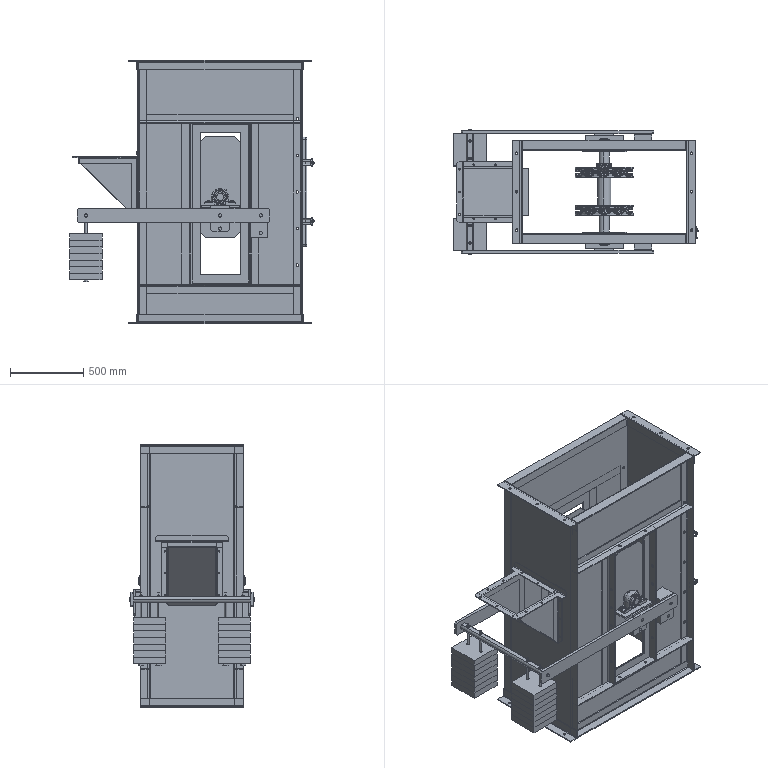Assembly | SolidWorks | mm | 60 component files | 82 solids | 3008 faces | box 1670 x 856 x 1800 mm | volume 98350600 mm3 | plane 1018 | cylinder 784 | cone 482 | sphere 288 | torus 282 | spline 154 | commonest cylinder face diameters 18 x195 20 x67 12 x62 367 x52 9 x40 10 x34 22 x32 60 x24
Bill of materials:
AccessDoor | 1 |  | Thin rectangular panel with rounded corners and edges, with two eyelet tabs sticking out from one long edge and two small hooked/slotted tabs on the face near the opposite edge.
ConnectingRod | 2 |  | Long, flat rectangular bar with chamfered corners and three small through holes along its centerline, spaced unevenly.
Counterweight | 14 |  | Square, fairly thick plate or block with two round through holes on one centerline.
FixedFrame | 1 |  | Long shaft with two parallel flats along its main body, smaller round journals at both ends, and four radial holes through the flat face.
GB_T62.1-2004WingNutRoundWingM12_1.75 | 2 |  | Bent bracket or lug with a central cylindrical boss with a through bore, and two angled arms that end in rounded eyelets with holes.
GuideFrame_2 | 2 |  | Open rectangular frame made of flat-bar members set on edge, with small holes along its sides and ends.
HangerRod | 4 |  | Long, slender cylindrical rod with a thin hexagonal head at one end and a short, smaller-diameter stepped pin at the other end.
hex nuts 1-fine pitch-grades ab gb | 8 |  | Hexagonal nut-shaped block with a central round through bore and chamfered corners on both faces.
Inlet | 1 |  | Sheet-metal chute or hopper: a rectangular flanged inlet frame with bolt holes, a sloped bottom wall, triangular side walls, and flanged side strips with holes.
LinkBolt | 2 |  | Lever-type part: a short cylindrical ring boss with a through bore and a straight cylindrical arm sticking out sideways, ending in a chamfered tip.
LowerCasing | 1 |  | Sheet-metal rectangular box housing with flanged top and bottom openings that have bolt holes, inner reinforcing channels or ribs, a rectangular side window, a rectangular opening in the back panel, and small lugs and a small block attached.
curved single coil spring lock washers gb | 4 |  | Flat split ring with a rectangular cross-section and a single radial gap.
DriveSprocket-Driven2 | 1 |  | Disc-shaped wheel with a groove around the rim, a raised central hub with a keyed bore, and six round lightening holes in a ring around the web; resembles a grooved pulley or sheave.
DriveSprocket-DrivenWithBearingHole2 | 1 |  | Disc-shaped grooved wheel almost identical to the keyed variant, but with a plain round central bore inside a raised hub, and six round holes in the web.
GB_T276-94[DeepGrooveBallBearing61914-2Z]2 | 2 |  | Flat annular part made of an outer ring and an inner ring separated by a narrow gap that holds evenly spaced small elements; resembles a thin-section rolling bearing.
GB_T7810-1995BearingWithVerticalSeatUELP210 | 2 |  | Housing on a pedestal base: a rectangular base with two elongated mounting holes supports a rounded, arch-shaped housing. The housing holds a ring insert with a round bore, and a small nipple-like stub sits on top; resembles a pillow-block bearing unit.
GB_T812-1988[RoundNutM68_2] | 2 |  | Flat thick ring with four rectangular notches evenly spaced around the outer edge and chamfered outer edges; resembles a slotted ring nut or locknut.
GB858-1988[LockWasherForRoundNut68_1.5]-Driven2 | 1 |  | Thin flat washer-like ring with one tab pointing inward from the bore edge and several rectangular tabs pointing outward around the outer edge. Some outer tabs are bent out of plane; resembles a tab lock washer.
GuideFrame | 2 |  | L-shaped (angle) bracket of flat plate: a wide horizontal flange with two round holes, joined at right angles to a narrower leg with two round holes and chamfered free corners.
hexagon head bolts--product grade c gb | 4 |  | Hexagon-head fastener-like part: a hexagonal head with a round bearing face and a plain cylindrical shank with a chamfered end; resembles a hex bolt or screw.
LowerAxis | 1 |  | Stepped cylindrical shaft with a larger central section and several smaller-diameter steps toward each end, plus a possible keyway or flat on one step.
ProtectivePlate | 2 |  | Very thin flat rectangular plate with chamfered corners and one central round hole; resembles a shim or spacer plate.
Mates:
1. coincident | LowerCasing-1 face at (-563, -290, 900) dir (-1, 0, 0) | Inlet-1 face at (-563, -163, -195) dir (1, 0, 0)
2. parallel | LowerCasing-1 face at (-563, -290, 900) dir (0, -1, 0) | Inlet-1 face at (-762, -163, 240) dir (0, -1, 0)
3. parallel | ConnectingRod-1 face at (-977, -398, -110) dir (0, 0, 1) | ConnectingRod-2 face at (-977, 418, -110) dir (0, 0, 1)
4. concentric | ConnectingRod-1 face at (-917, -398, -160) dir (0, -1, 0) r 11 | ConnectingRod-2 face at (-917, 418, -160) dir (0, -1, 0) r 11
5. width | ConnectingRod-1 face at (-319.5, -418, -160) dir (0, -1, 0) | ConnectingRod-2 face at (-319.5, 418, -160) dir (0, 1, 0) | LowerCasing-1 face at (-563, 290, 900) dir (0, 1, 0) | LowerCasing-1 face at (-563, -290, 900) dir (0, -1, 0)
6. distance | ConnectingRod-2 face at (-319.5, 398, -160) dir (0, -1, 0) | ConnectingRod-1 face at (-319.5, -398, -160) dir (0, 1, 0)
7. parallel | LowerCasing-1 face at (-652.095, -290, -630) dir (0, 0, 1) | ConnectingRod-1 face at (-977, -398, -110) dir (0, 0, 1)
8. distance | ConnectingRod-1 sketch segment at (278, -409.25, -160) dir (0, -1, 0) | LowerCasing-1 face at (563, -290, 900) dir (1, 0, 0)
9. distance | ConnectingRod-1 sketch segment at (278, -409.25, -160) dir (0, -1, 0) | LowerCasing-1 face at (563, 353, -900) dir (0, 0, -1)
10. concentric | ConnectingRod-2 face at (-917, 418, -160) dir (0, -1, 0) r 11 | FixedFrame-1 face at (-917, -428, -160) dir (0, 1, 0) r 11
11. coincident | ConnectingRod-1 face at (-319.5, -398, -160) dir (0, 1, 0) | FixedFrame-1 face at (-917, -398, -160) dir (0, -1, 0)
12. parallel | ConnectingRod-2 face at (-977, 418, -110) dir (0, 0, 1) | FixedFrame-1 face at (-947, 428, -140) dir (0, 0, 1)
13. concentric | FixedFrame-1 face at (-917, 348, -796) dir (0, 0, 1) r 9 | HangerRod-1 face at (-917, 348, -115) dir (0, 0, -1) r 8
14. distance | HangerRod-1 face at (-917, 348, -115) dir (0, 0, 1) | FixedFrame-1 face at (-947, 428, -140) dir (0, 0, 1)
15. concentric | FixedFrame-1 face at (-917, 228, -796) dir (0, 0, 1) r 9 | HangerRod-2 face at (-917, 228, -115) dir (0, 0, -1) r 8
16. coincident | HangerRod-1 face at (-917, 348, -115) dir (0, 0, 1) | HangerRod-2 face at (-917, 228, -115) dir (0, 0, 1)
17. concentric | Counterweight-1 face at (-917, 348, -555) dir (0, 0, -1) r 10 | HangerRod-1 face at (-917, 348, -115) dir (0, 0, -1) r 8
18. concentric | Counterweight-1 edge at (-917, 228, -555) dir (0, 0, 1) r 10 | HangerRod-2 face at (-917, 228, -115) dir (0, 0, -1) r 8
19. coincident | Counterweight-1 face at (-917, 288, -600) dir (0, 0, -1) | HangerRod-1 face at (-917, 348, -600) dir (0, 0, 1)
20. concentric | FixedFrame-1 face at (-917, 228, -796) dir (0, 0, 1) r 9 | hex nuts 1-fine pitch-grades ab gb-2 face at (-917, 228, -140) dir (0, 0, 1) r 523.599
21. coincident | FixedFrame-1 face at (-947, 428, -140) dir (0, 0, 1) | hex nuts 1-fine pitch-grades ab gb-2 face at (-930.856, 220, -140) dir (0, 0, -1)
22. concentric | FixedFrame-1 face at (-917, 348, -796) dir (0, 0, 1) r 9 | hex nuts 1-fine pitch-grades ab gb-3 face at (-917, 348, -140) dir (0, 0, 1) r 523.599
23. coincident | FixedFrame-1 face at (-947, 428, -140) dir (0, 0, 1) | hex nuts 1-fine pitch-grades ab gb-3 face at (-930.856, 340, -140) dir (0, 0, -1)
24. coincident | LowerCasing-1 face at (-652.095, -290, -630) dir (0, 0, 1) | GuideFrame_2-1 face at (-200, -353, -630) dir (0, 0, -1)
25. coincident | LowerCasing-1 face at (200, -353, -500000) dir (-1, 0, 0) | GuideFrame_2-1 face at (200, -353, -630) dir (1, 0, 0)
26. coincident | LowerCasing-1 face at (-563, -290, 900) dir (0, -1, 0) | GuideFrame_2-1 face at (0, -290, -80) dir (0, 1, 0)
27. concentric | LowerTensioningDeviceAssembly-1/GuideFrame-2 face at (0, -398, -160) dir (0, 1, 0) r 11 | ConnectingRod-1 face at (0, -398, -160) dir (0, -1, 0) r 11
28. coincident | LowerTensioningDeviceAssembly-1/GuideFrame-2 face at (65, -398, -95) dir (0, -1, 0) | ConnectingRod-1 face at (-319.5, -398, -160) dir (0, 1, 0)
29. perpendicular | LowerTensioningDeviceAssembly-1/GuideFrame-1 face at (-65, 74, -270) dir (-1, 0, 0) | ConnectingRod-2 face at (-977, 418, -110) dir (0, 0, 1)
30. coincident | LowerCasing-1 face at (563, -290, 900) dir (1, 0, 0) | AccessDoor-1 face at (563, -269, -357) dir (-1, 0, 0)
31. parallel | LowerCasing-1 edge at (563, -200, 350) dir (0, 0, -1) | AccessDoor-1 edge at (563, -289, 357) dir (0, 0, -1)
32. width | AccessDoor-1 face at (563, -269, 377) dir (0.1736, 0, 0.9848) | AccessDoor-1 face at (563, -269, -377) dir (0.1736, 0, -0.9848) | LowerCasing-1 face at (553, -200, 350) dir (0, 0, -1) | LowerCasing-1 face at (553, -200, -350) dir (0, 0, 1)
33. width | AccessDoor-1 face at (563, -289, -357) dir (0.1736, -0.9848, 0) | AccessDoor-1 face at (563, 289, -357) dir (0.1736, 0.9848, 0) | LowerCasing-1 face at (553, -200, 350) dir (0, 1, 0) | LowerCasing-1 face at (553, 200, 350) dir (0, -1, 0)
34. concentric | AccessDoor-1 face at (628, -219, 200) dir (0, -1, 0) r 6.5 | LinkBolt-1 face at (628, -243, 200) dir (0, -1, 0) r 6
35. concentric | LowerCasing-1 face at (628, -313, 205) dir (0, 0, -1) r 5 | LinkBolt-1 face at (628, -313, 207) dir (0, 0, -1) r 8
36. concentric | LowerCasing-1 face at (628, -313, -205) dir (0, 0, 1) r 5 | LinkBolt-2 face at (628, -313, -193) dir (0, 0, -1) r 8
37. concentric | AccessDoor-1 face at (628, -219, -200) dir (0, -1, 0) r 6.5 | LinkBolt-2 face at (628, -243, -200) dir (0, -1, 0) r 6
38. concentric | LinkBolt-1 face at (628, -243, 200) dir (0, -1, 0) r 6 | GB_T62.1-2004WingNutRoundWingM12_1.75-1 face at (628, -234, 200) dir (0, -1, 0) r 6
39. coincident | AccessDoor-1 face at (643, -261, 215) dir (0, 1, 0) | GB_T62.1-2004WingNutRoundWingM12_1.75-1 face at (628, -261, 200) dir (0, -1, 0)
40. concentric | LinkBolt-2 face at (628, -243, -200) dir (0, -1, 0) r 6 | GB_T62.1-2004WingNutRoundWingM12_1.75-2 face at (628, -234, -200) dir (0, -1, 0) r 6
41. coincident | AccessDoor-1 face at (643, -261, -215) dir (0, 1, 0) | GB_T62.1-2004WingNutRoundWingM12_1.75-2 face at (628, -261, -200) dir (0, -1, 0)
42. parallel | LowerCasing-1 face at (563, -290, 989.095) dir (1, 0, 0) | GB_T62.1-2004WingNutRoundWingM12_1.75-2 face at (626, -242.5, -220.5) dir (-1, 0, 0)
43. parallel | LowerCasing-1 face at (563, -290, 989.095) dir (1, 0, 0) | GB_T62.1-2004WingNutRoundWingM12_1.75-1 face at (626, -242.5, 179.5) dir (-1, 0, 0)
44. concentric | LowerCasing-1 face at (-300, -263, 900) dir (0, 0, -1) r 9 | assembly face at (-300, -263, 927) dir (0, 0, -1) r 8
45. coincident | LowerCasing-1 face at (652.095, -303, 892) dir (0, 0, -1) | assembly face at (-288.165, -269.833, 892) dir (0, 0, 1)
46. concentric | LowerCasing-1 face at (-598, -263, 900) dir (0, 0, -1) r 9 | assembly face at (-598, -263, 916) dir (0, 0, 1) r 8
47. coincident | LowerCasing-1 face at (-626, 353, 894) dir (0, 0, -1) | assembly face at (-598, -263, 894) dir (0, 0, 1)
48. coincident | LowerCasing-1 face at (652.095, -303, 892) dir (0, 0, -1) | assembly face at (-300, -263, 892) dir (0, 0, 1)
49. coincident | assembly face at (-300, -263, 869) dir (0, 0, -1) | assembly face at (0, -263, 869) dir (0, 0, -1)
50. coincident | assembly face at (0, -263, 869) dir (0, 0, -1) | assembly face at (300, -263, 869) dir (0, 0, -1)
51. concentric | LowerCasing-1 face at (598, -263, 900) dir (0, 0, -1) r 9 | assembly face at (598, -263, 914) dir (0, 0, 1) r 8
52. coincident | assembly face at (300, -263, 869) dir (0, 0, -1) | assembly face at (598, -263, 869) dir (0, 0, -1)
53. concentric | LowerCasing-1 face at (598, 0, 900) dir (0, 0, -1) r 9 | assembly face at (598, 0, 914) dir (0, 0, 1) r 8
54. coincident | assembly face at (598, -263, 869) dir (0, 0, -1) | assembly face at (598, 0, 869) dir (0, 0, -1)
55. concentric | LowerCasing-1 face at (598, 263, 900) dir (0, 0, -1) r 9 | assembly face at (598, 263, 914) dir (0, 0, 1) r 8
56. coincident | assembly face at (598, 263, 869) dir (0, 0, -1) | assembly face at (598, 0, 869) dir (0, 0, -1)
57. concentric | LowerCasing-1 face at (-598, 263, 900) dir (0, 0, -1) r 9 | assembly face at (-598, 263, 916) dir (0, 0, 1) r 8
58. concentric | LowerCasing-1 face at (-598, 0, 900) dir (0, 0, -1) r 9 | assembly face at (-598, 0, 916) dir (0, 0, 1) r 8
59. coincident | assembly face at (-598, -263, 871) dir (0, 0, -1) | assembly face at (-598, 263, 871) dir (0, 0, -1)
60. coincident | assembly face at (-598, -263, 871) dir (0, 0, -1) | assembly face at (-598, 0, 871) dir (0, 0, -1)
61. coincident | assembly face at (-300, 263, 871) dir (0, 0, -1) | assembly face at (-598, 263, 871) dir (0, 0, -1)
62. coincident | assembly face at (0, 263, 871) dir (0, 0, -1) | assembly face at (-300, 263, 871) dir (0, 0, -1)
63. coincident | assembly face at (300, 263, 871) dir (0, 0, -1) | assembly face at (0, 263, 871) dir (0, 0, -1)
64. concentric | LowerAxis-1 face at (0, 0, -364) dir (0, 0, 1) r 25 | GB_T7810-1995BearingWithVerticalSeatUELP210-1 face at (0, 0, -320.6) dir (0, 0, -1) r 25
65. coincident | LowerAxis-1 face at (0, 0, -296) dir (0, 0, -1) | GB_T7810-1995BearingWithVerticalSeatUELP210-1 face at (-32.817, 3.473, -296) dir (0, 0, 1)
66. concentric | LowerAxis-1 face at (0, 0, 364) dir (0, 0, -1) r 25 | GB_T7810-1995BearingWithVerticalSeatUELP210-2 face at (0, 0, 320.6) dir (0, 0, 1) r 25
67. coincident | LowerAxis-1 face at (0, 0, 296) dir (0, 0, 1) | GB_T7810-1995BearingWithVerticalSeatUELP210-2 face at (-32.817, 3.473, 296) dir (0, 0, -1)
68. parallel | GB_T7810-1995BearingWithVerticalSeatUELP210-1 face at (30.336, -38.309, -338.9) dir (-0.9944, 0.1053, 0) | GB_T7810-1995BearingWithVerticalSeatUELP210-2 face at (30.336, -38.309, 338.9) dir (-0.9944, 0.1053, 0)
69. coincident | GB_T7810-1995BearingWithVerticalSeatUELP210-1 face at (53.209, -40.73, -351.1) dir (0.9944, -0.1053, 0) | GuideFrame-1 face at (43.199, -135.298, -384) dir (-0.9944, 0.1053, 0)
70. width | GuideFrame-1 face at (229.041, -89.605, -74) dir (-0.1053, -0.9944, 0) | GuideFrame-1 face at (242.724, 39.673, -74) dir (0.1053, 0.9944, 0) | GB_T7810-1995BearingWithVerticalSeatUELP210-1 face at (50.446, 99.242, -351.1) dir (0.1053, 0.9944, 0) | GB_T7810-1995BearingWithVerticalSeatUELP210-1 face at (28.553, -107.603, -351.1) dir (-0.1053, -0.9944, 0)
71. distance | GuideFrame-1 face at (55.013, -71.186, -398) dir (0, 0, -1) | GB_T7810-1995BearingWithVerticalSeatUELP210-1 face at (53.209, -40.73, -351.1) dir (0, 0, -1)
72. concentric | GuideFrame-1 face at (65.25, 73.038, -320.6) dir (-0.9944, 0.1053, 0) r 9 | hexagon head bolts--product grade c gb-1 face at (44.366, 75.248, -320.6) dir (0.9944, -0.1053, 0) r 4
73. coincident | GuideFrame-1 face at (57.122, -136.772, -384) dir (0.9944, -0.1053, 0) | hexagon head bolts--product grade c gb-1 face at (79.222, 72.035, -328.091) dir (-0.9944, 0.1053, 0)
74. concentric | GuideFrame-1 face at (48.515, -85.079, -320.6) dir (-0.9944, 0.1053, 0) r 9 | hexagon head bolts--product grade c gb-2 face at (27.631, -82.869, -320.6) dir (0.9944, -0.1053, 0) r 4
75. coincident | GuideFrame-1 face at (57.122, -136.772, -384) dir (0.9944, -0.1053, 0) | hexagon head bolts--product grade c gb-2 face at (62.487, -86.082, -328.091) dir (-0.9944, 0.1053, 0)
76. coincident | GB_T7810-1995BearingWithVerticalSeatUELP210-1 face at (30.336, -38.309, -338.9) dir (-0.9944, 0.1053, 0) | curved single coil spring lock washers gb-4 face at (25.642, -82.658, -320.6) dir (0.9944, -0.1053, 0)
77. concentric | hexagon head bolts--product grade c gb-2 face at (27.631, -82.869, -320.6) dir (0.9944, -0.1053, 0) r 4 | curved single coil spring lock washers gb-4 face at (25.642, -82.658, -320.6) dir (-0.9944, 0.1053, 0) r 2.1
78. concentric | hexagon head bolts--product grade c gb-1 face at (44.366, 75.248, -320.6) dir (0.9944, -0.1053, 0) r 4 | curved single coil spring lock washers gb-8 face at (42.378, 75.459, -320.6) dir (-0.9944, 0.1053, 0) r 1.5
79. coincident | GB_T7810-1995BearingWithVerticalSeatUELP210-1 face at (37.684, 31.11, -338.9) dir (-0.9944, 0.1053, 0) | curved single coil spring lock washers gb-8 face at (42.378, 75.459, -320.6) dir (0.9944, -0.1053, 0)
80. concentric | curved single coil spring lock washers gb-4 face at (25.642, -82.658, -320.6) dir (-0.9944, 0.1053, 0) r 1.5 | hex nuts 1-fine pitch-grades ab gb-2 face at (25.046, -82.595, -320.6) dir (-0.9944, 0.1053, 0) r 523.599
81. coincident | curved single coil spring lock washers gb-4 face at (25.046, -82.595, -320.6) dir (-0.9944, 0.1053, 0) | hex nuts 1-fine pitch-grades ab gb-2 face at (23.454, -97.633, -325.826) dir (0.9944, -0.1053, 0)
82. concentric | curved single coil spring lock washers gb-8 face at (42.378, 75.459, -320.6) dir (-0.9944, 0.1053, 0) r 1.5 | hex nuts 1-fine pitch-grades ab gb-3 face at (41.781, 75.522, -320.6) dir (-0.9944, 0.1053, 0) r 523.599
83. coincident | curved single coil spring lock washers gb-8 face at (41.781, 75.522, -320.6) dir (-0.9944, 0.1053, 0) | hex nuts 1-fine pitch-grades ab gb-3 face at (40.189, 60.483, -325.826) dir (0.9944, -0.1053, 0)
84. width | ProtectivePlate-1 face at (291.448, 119.991, 280.1) dir (0.1053, 0.9944, 0) | ProtectivePlate-1 face at (259.872, -178.343, 280.1) dir (-0.1053, -0.9944, 0) | GuideFrame-2 face at (242.724, 39.673, 74) dir (0.1053, 0.9944, 0) | GuideFrame-2 face at (229.041, -89.605, 74) dir (-0.1053, -0.9944, 0)
85. coincident | GuideFrame-2 face at (222.2, -154.244, 280.1) dir (0, 0, -1) | ProtectivePlate-1 face at (-67.423, 7.136, 280.1) dir (0, 0, 1)
86. distance | ProtectivePlate-1 edge at (265.135, -128.621, 280.1) dir (0.1053, 0.9944, 0) | GuideFrame-2 face at (70.565, 123.257, 384) dir (-0.9944, 0.1053, 0)
87. concentric | LowerAxis-1 face at (0, 0, 160) dir (0, 0, -1) r 35 | DriveSprocket-DrivenWithBearingHole2-1 face at (0, 0, -116) dir (0, 0, 1) r 50
88. coincident | LowerAxis-1 edge at (0, 0, -98) dir (0, 0, 1) r 45 | DriveSprocket-DrivenWithBearingHole2-1 face at (13.738, 198.024, -98) dir (0, 0, 1)
89. concentric | DriveSprocket-DrivenWithBearingHole2-1 face at (0, 0, -116) dir (0, 0, 1) r 50 | GB_T276-94[DeepGrooveBallBearing61914-2Z]2-1 face at (0, 0, -93.579) dir (0, 0, 1) r 35
90. coincident | LowerAxis-1 edge at (0, 0, -98) dir (0, 0, 1) r 45 | GB_T276-94[DeepGrooveBallBearing61914-2Z]2-1 face at (0, 49, -98) dir (0, 0, 1)
91. concentric | DriveSprocket-DrivenWithBearingHole2-1 face at (0, 0, -150) dir (0, 0, -1) r 50 | GB_T276-94[DeepGrooveBallBearing61914-2Z]2-2 face at (0, 0, -158) dir (0, 0, 1) r 50
92. coincident | DriveSprocket-DrivenWithBearingHole2-1 face at (0, 0, -150) dir (0, 0, -1) | GB_T276-94[DeepGrooveBallBearing61914-2Z]2-2 face at (0, 49, -150) dir (0, 0, 1)
93. concentric | LowerAxis-1 face at (0, 0, 160) dir (0, 0, -1) r 35 | DriveSprocket-Driven2-1 face at (0, 0, 90) dir (0, 0, 1) r 35
94. coincident | LowerAxis-1 face at (0, 0, 90) dir (0, 0, 1) | DriveSprocket-Driven2-1 face at (-197.176, 22.892, 90) dir (0, 0, -1)
95. concentric | LowerAxis-1 face at (0, 0, -296) dir (0, 0, 1) r 34 | GB_T812-1988[RoundNutM68_2]-1 face at (0, 0, -168) dir (0, 0, -1) r 34
96. coincident | DriveSprocket-DrivenWithBearingHole2-1 face at (13.738, 198.024, -168) dir (0, 0, -1) | GB_T812-1988[RoundNutM68_2]-1 face at (0, 0, -168) dir (0, 0, 1)
97. coincident | GB_T812-1988[RoundNutM68_2]-1 face at (0, 0, -180) dir (0, 0, -1) | GB858-1988[LockWasherForRoundNut68_1.5]-Driven2-1 face at (0, 44, -180) dir (0, 0, 1)
98. concentric | LowerAxis-1 face at (0, 0, -296) dir (0, 0, 1) r 34 | GB858-1988[LockWasherForRoundNut68_1.5]-Driven2-1 face at (0, 0, -185.465) dir (0, 0, 1) r 34.5
99. concentric | LowerAxis-1 face at (0, 0, -296) dir (0, 0, 1) r 34 | GB_T812-1988[RoundNutM68_2]-2 face at (0, 0, -193.5) dir (0, 0, 1) r 34
100. coincident | GB858-1988[LockWasherForRoundNut68_1.5]-Driven2-1 face at (0, 44, -181.5) dir (0, 0, -1) | GB_T812-1988[RoundNutM68_2]-2 face at (0, 0, -181.5) dir (0, 0, 1)